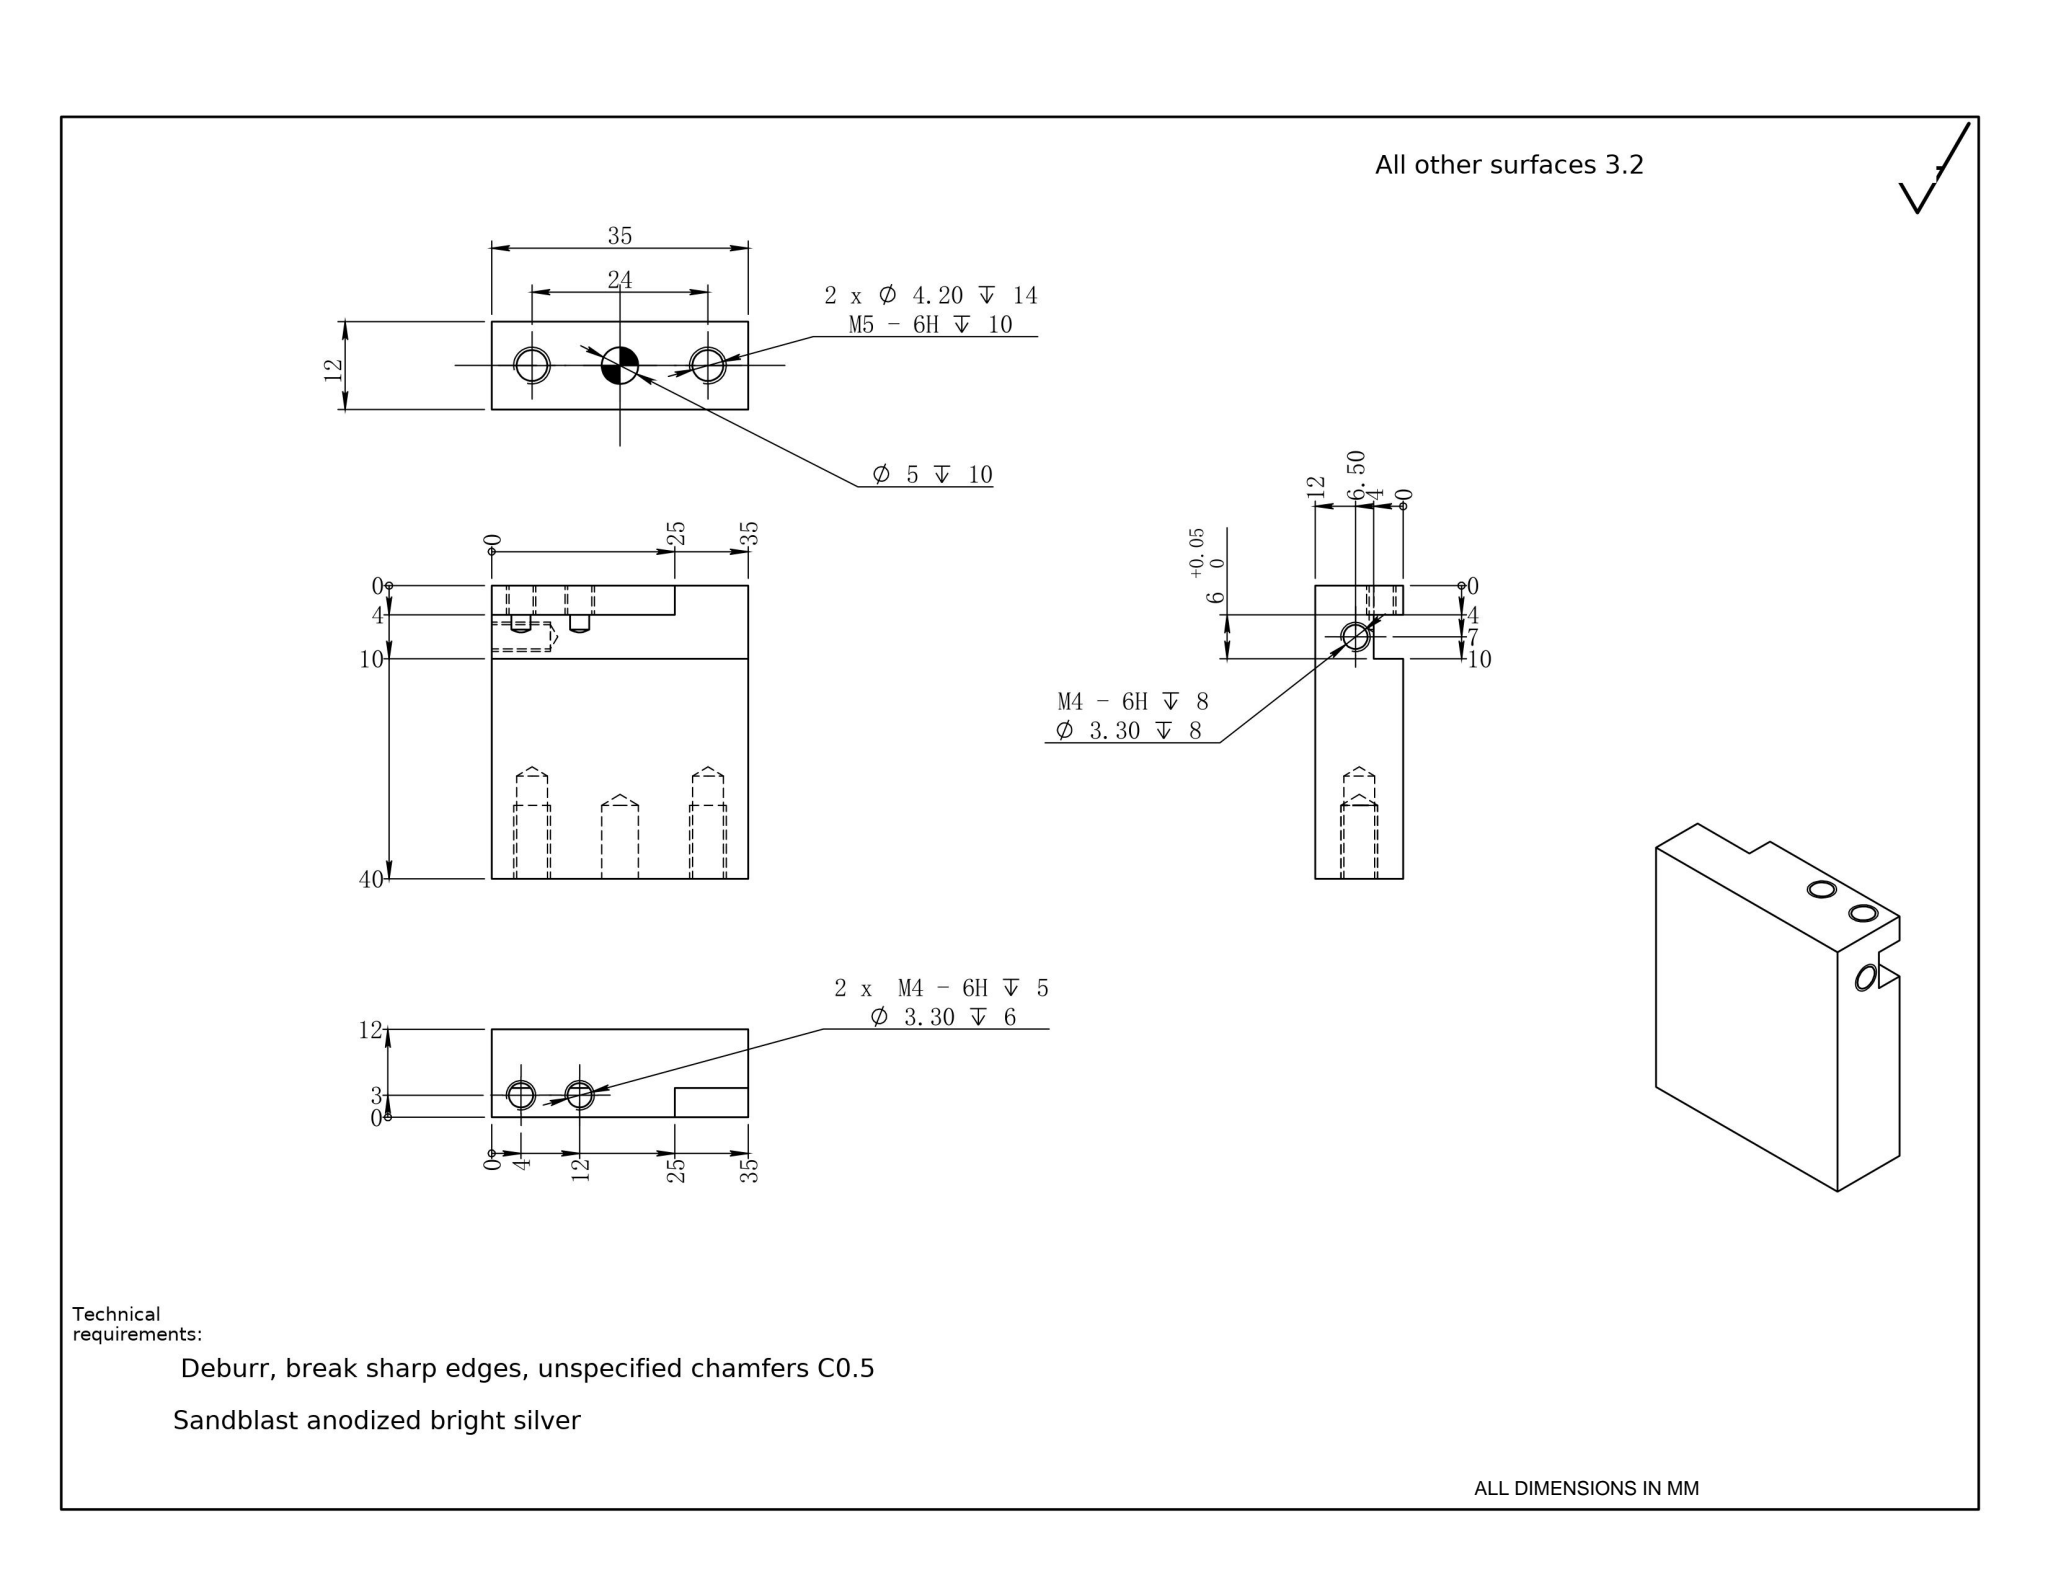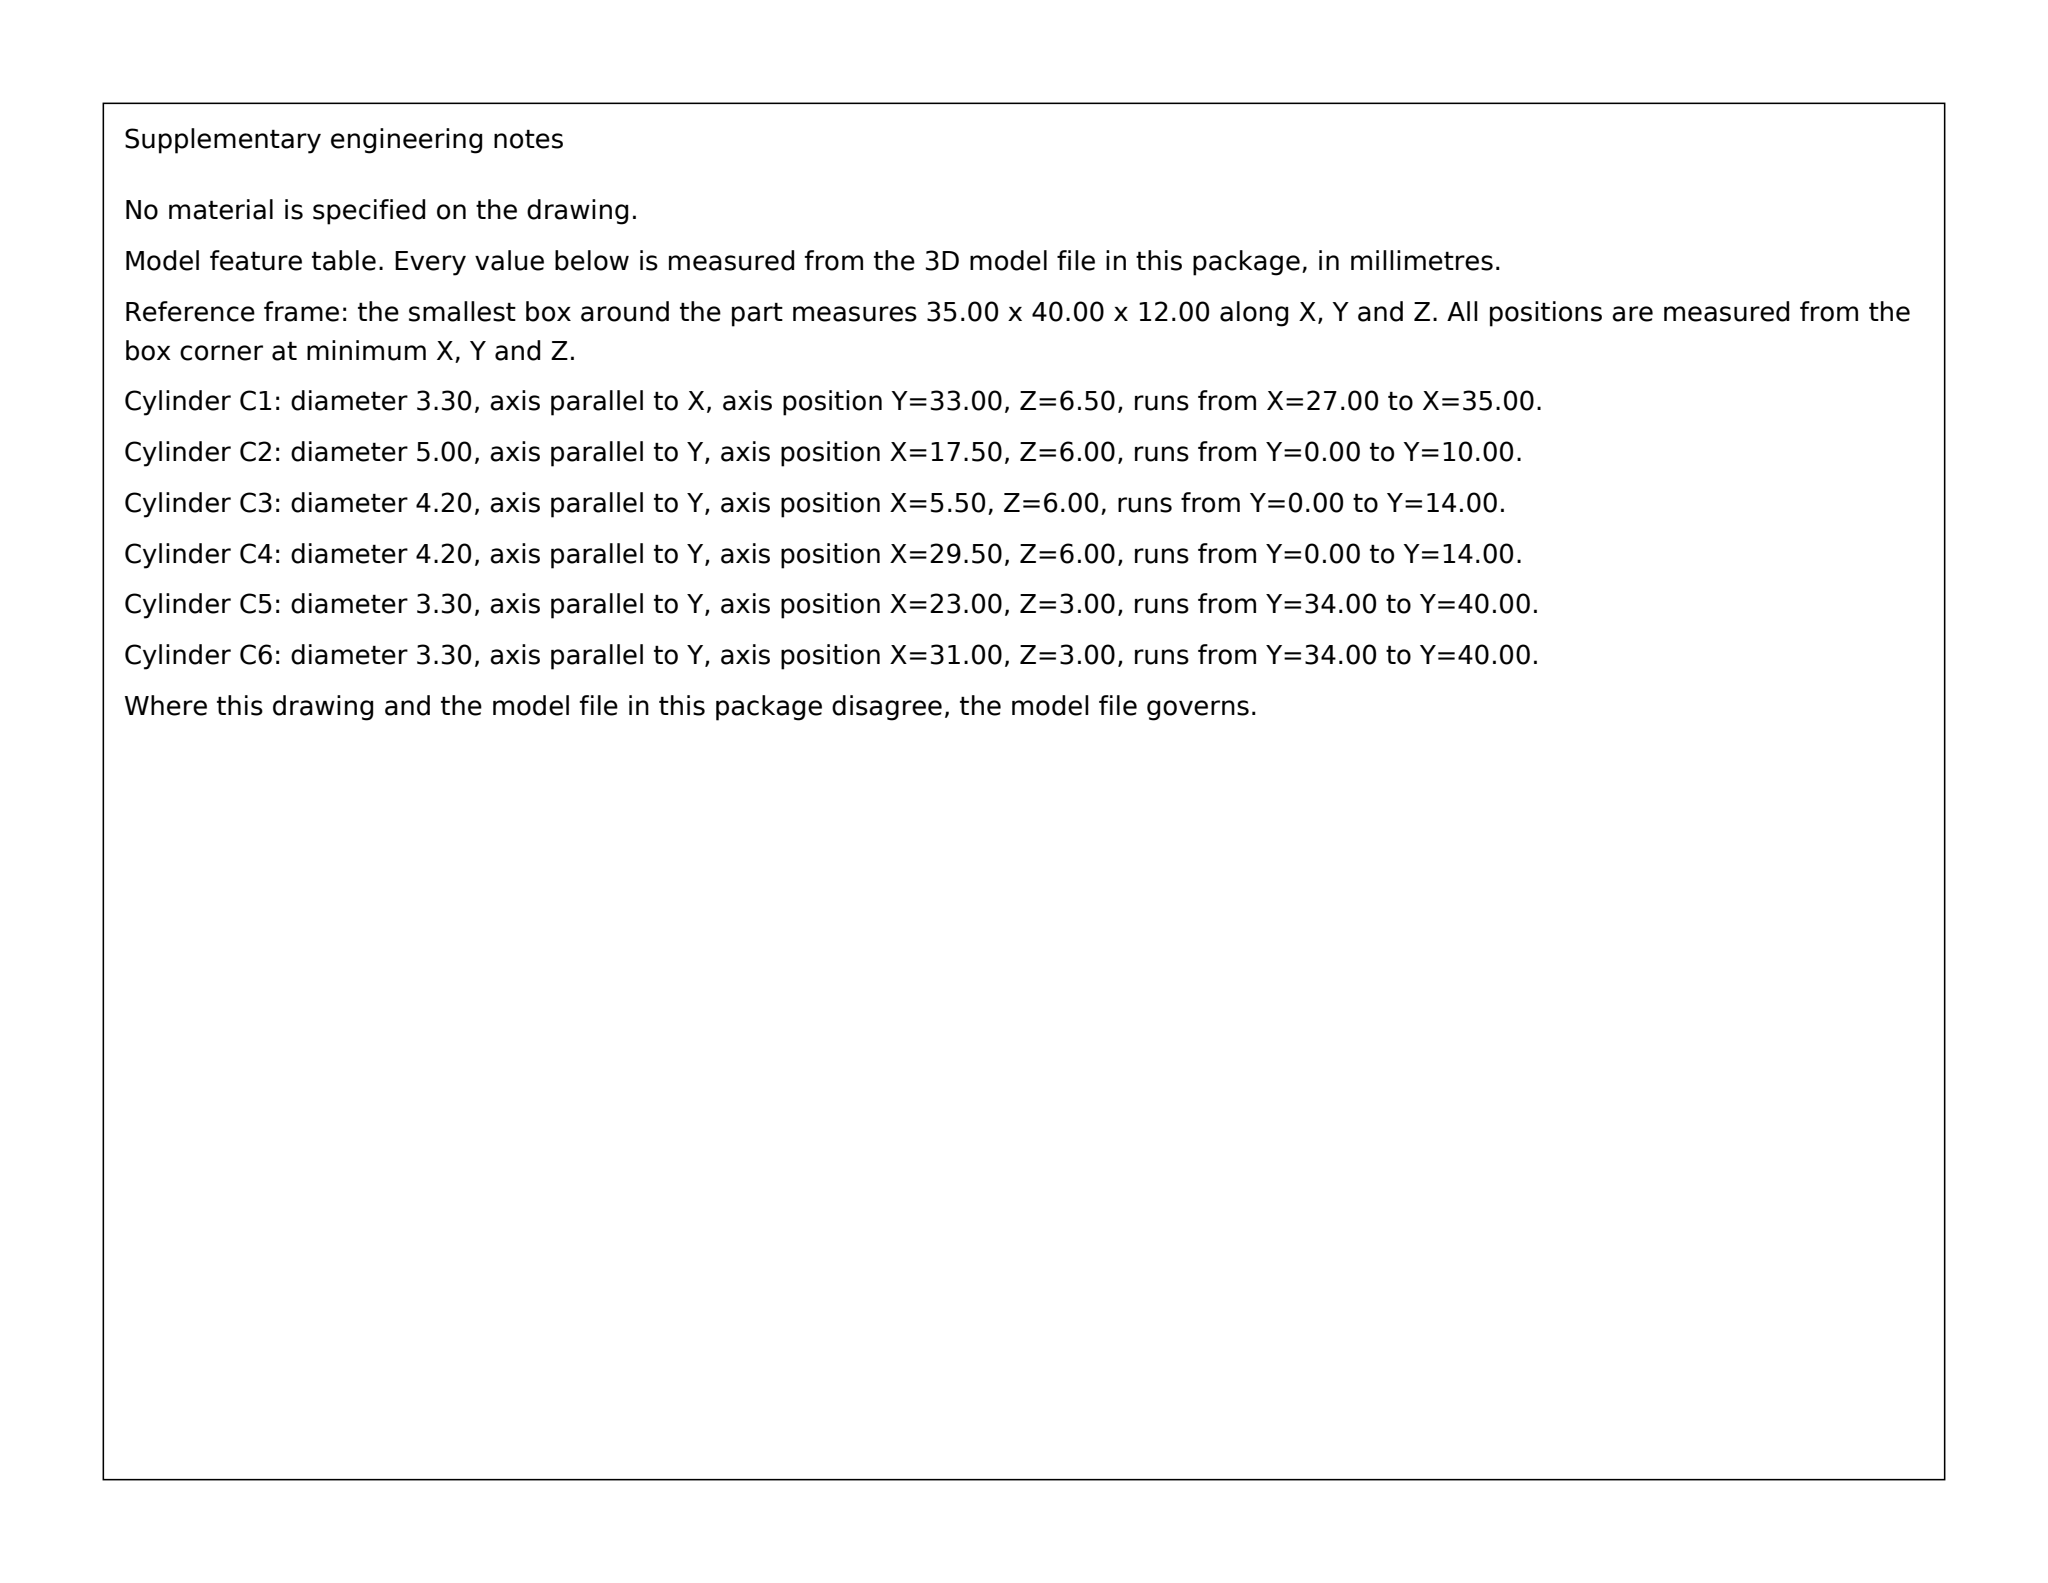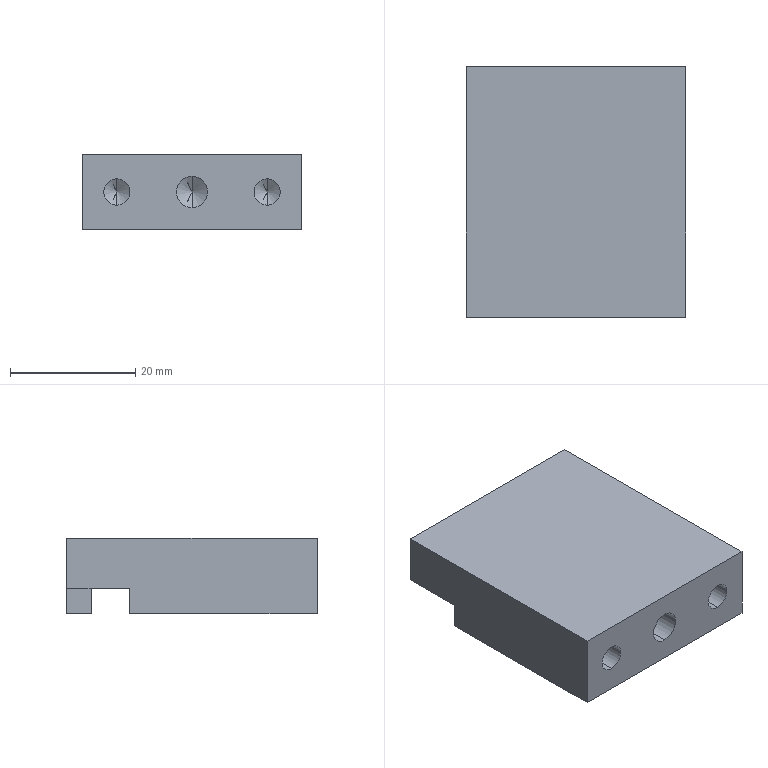Part | SolidWorks | mm | 1 solid | 35 faces | box 35 x 40 x 12 mm | volume 15049 mm3 | cylinder 12 | cone 12 | plane 11 | commonest cylinder face diameters 3.3 x6 4.2 x4 5 x2
build123d program:
from build123d import *

# Parameters (mm, degrees)
SKETCH1_W                    = 35
SKETCH1_H                    = 40
BOSS_EXTRUDE1_DEPTH          = 6
SKETCH2_W                    = 8
SKETCH2_H                    = 6
CUT_EXTRUDE1_DEPTH           = 54.488
SKETCH11_W                   = 10
SKETCH11_H                   = 4
CUT_EXTRUDE2_DEPTH           = 5
M4_TAPPED_HOLE1_D            = 3.3
M4_TAPPED_HOLE1_DEPTH        = 8
M4_TAPPED_HOLE1_TIP          = 0.9914
M4_TAPPED_HOLE2_D            = 3.3
M4_TAPPED_HOLE2_DEPTH        = 6
M4_TAPPED_HOLE2_TIP          = 0.9914
M5_TAPPED_HOLE1_D            = 4.2
M5_TAPPED_HOLE1_DEPTH        = 14
M5_TAPPED_HOLE1_TIP          = 1.262
F_5_0_5_DIAMETER_HOLE1_D     = 5
F_5_0_5_DIAMETER_HOLE1_DEPTH = 10
F_5_0_5_DIAMETER_HOLE1_TIP   = 1.502


with BuildPart() as part:
    # Sketch1 → Boss-Extrude1 (new, symmetric)
    with BuildSketch(Plane.XY):
        with Locations((0, 20)):
            Rectangle(SKETCH1_W, SKETCH1_H)
    extrude(amount=BOSS_EXTRUDE1_DEPTH, both=True)

    # Sketch2 → Cut-Extrude1 (cut, through all)
    with BuildSketch(Plane(origin=(17.5, 0, 0), x_dir=(0, 0, -1), z_dir=(1, 0, 0))):
        with Locations((6, 33)):
            Rectangle(SKETCH2_W, SKETCH2_H)
    extrude(amount=-CUT_EXTRUDE1_DEPTH, mode=Mode.SUBTRACT)

    # Sketch11 → Cut-Extrude2 (cut)
    with BuildSketch(Plane(origin=(0, 40, 0), x_dir=(1, 0, 0), z_dir=(0, 1, 0))):
        with Locations((-12.5, 4)):
            Rectangle(SKETCH11_W, SKETCH11_H)
    extrude(amount=-CUT_EXTRUDE2_DEPTH, mode=Mode.SUBTRACT)

    # M4 Tapped Hole1
    with Locations(Plane(origin=(17.5, -12.595, -3.067), x_dir=(0, 0, 1), z_dir=(1, 0, 0))):
        with Locations((3.567, -45.595)):
            Hole(M4_TAPPED_HOLE1_D / 2, depth=M4_TAPPED_HOLE1_DEPTH)
            with Locations((0, 0, -(M4_TAPPED_HOLE1_DEPTH + M4_TAPPED_HOLE1_TIP / 2))):  # 118° drill point
                Cone(0, M4_TAPPED_HOLE1_D / 2, M4_TAPPED_HOLE1_TIP, mode=Mode.SUBTRACT)

    # M4 Tapped Hole2
    with Locations(Plane(origin=(0, 40, 0), x_dir=(1, 0, 0), z_dir=(0, 1, 0))):
        with Locations((5.5, 3), (13.5, 3)):
            Hole(M4_TAPPED_HOLE2_D / 2, depth=M4_TAPPED_HOLE2_DEPTH)
            with Locations((0, 0, -(M4_TAPPED_HOLE2_DEPTH + M4_TAPPED_HOLE2_TIP / 2))):  # 118° drill point
                Cone(0, M4_TAPPED_HOLE2_D / 2, M4_TAPPED_HOLE2_TIP, mode=Mode.SUBTRACT)

    # M5 Tapped Hole1
    with Locations(Plane(origin=(0, 0, 0), x_dir=(-1, 0, 0), z_dir=(0, -1, 0))):
        with Locations((-12, 0), (12, 0)):
            Hole(M5_TAPPED_HOLE1_D / 2, depth=M5_TAPPED_HOLE1_DEPTH)
            with Locations((0, 0, -(M5_TAPPED_HOLE1_DEPTH + M5_TAPPED_HOLE1_TIP / 2))):  # 118° drill point
                Cone(0, M5_TAPPED_HOLE1_D / 2, M5_TAPPED_HOLE1_TIP, mode=Mode.SUBTRACT)

    # 5.0 _5_ Diameter Hole1
    with Locations(Plane(origin=(0, 0, 0), x_dir=(-1, 0, 0), z_dir=(0, -1, 0))):
        with Locations((0, 0)):
            Hole(F_5_0_5_DIAMETER_HOLE1_D / 2, depth=F_5_0_5_DIAMETER_HOLE1_DEPTH)
            with Locations((0, 0, -(F_5_0_5_DIAMETER_HOLE1_DEPTH + F_5_0_5_DIAMETER_HOLE1_TIP / 2))):  # 118° drill point
                Cone(0, F_5_0_5_DIAMETER_HOLE1_D / 2, F_5_0_5_DIAMETER_HOLE1_TIP, mode=Mode.SUBTRACT)


solid = part.part